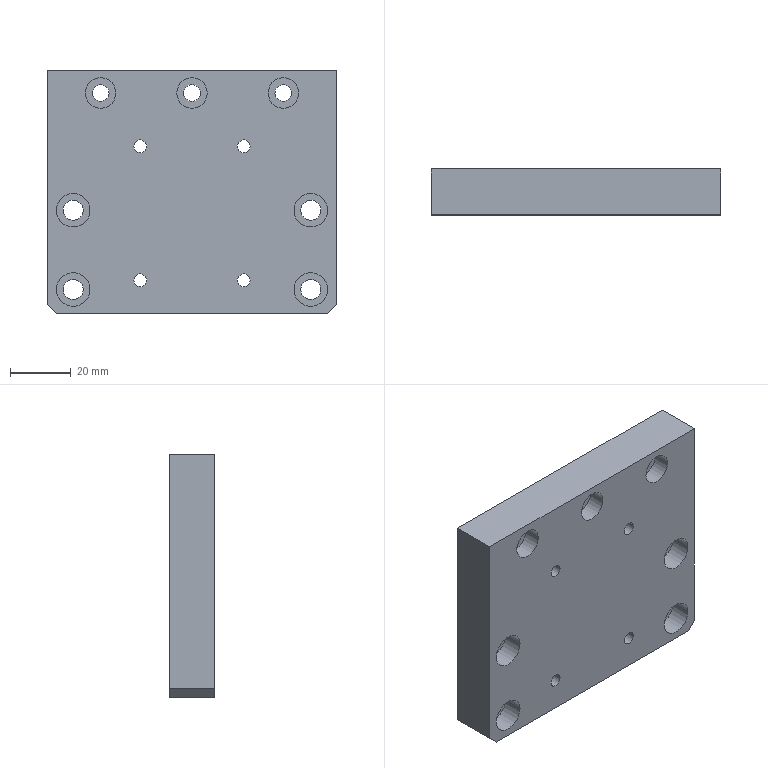Component | SolidWorks | LongSideClampingAssemblyBGeneralAssembly-1_FrameLowerPressPlateB-0510-1 | 1 solid | 51 faces | box 95 x 15 x 80 mm | volume 107321 mm3 | cylinder 36 | plane 15 | commonest cylinder face diameters 4.2 x8 11 x8 6.6 x8 10 x6 5.5 x6 | material Q235-A
build123d program:
from build123d import *

# Parameters (mm, degrees)
SKETCH1_W                                          = 95
SKETCH1_H                                          = 80
BOSS_EXTRUDE1_DEPTH                                = 15
CHAMFER1_SIZE                                      = 3
HOLE_SIZE_ACCORDING_TO_TYPE_OF_HEX_SOC_D           = 6.6
HOLE_SIZE_ACCORDING_TO_TYPE_OF_HEX_SOC_CBORE_D     = 11
HOLE_SIZE_ACCORDING_TO_TYPE_OF_HEX_SOC_CBORE_DEPTH = 6.8
M5_TAPPED_HOLE1_D                                  = 4.2
HOLE_SIZE_ACCORDING_TO_TYPE_OF_HEX_2_D             = 5.5
HOLE_SIZE_ACCORDING_TO_TYPE_OF_HEX_2_CBORE_D       = 10
HOLE_SIZE_ACCORDING_TO_TYPE_OF_HEX_2_CBORE_DEPTH   = 5.7


with BuildPart() as part:
    # Sketch1 → Boss-Extrude1 (new body)
    with BuildSketch(Plane.XY):
        with Locations((-47.5, 40)):
            Rectangle(SKETCH1_W, SKETCH1_H)
    extrude(amount=BOSS_EXTRUDE1_DEPTH)

    # Chamfer1
    chamfer1_edges = [part.edges().sort_by_distance(p)[0] for p in [
        (0, 0, 7.5),
        (-95, 0, 7.5),
    ]]
    chamfer(chamfer1_edges, length=CHAMFER1_SIZE)

    # Hole Size _According to_ Type of Hex Soc (through all)
    with Locations(Plane.XY.offset(15)):
        with Locations((-8.5, 8), (-86.5, 8), (-8.5, 34), (-86.5, 34)):
            CounterBoreHole(HOLE_SIZE_ACCORDING_TO_TYPE_OF_HEX_SOC_D / 2, HOLE_SIZE_ACCORDING_TO_TYPE_OF_HEX_SOC_CBORE_D / 2, HOLE_SIZE_ACCORDING_TO_TYPE_OF_HEX_SOC_CBORE_DEPTH)

    # M5 Tapped Hole1 (through all)
    with Locations(Plane.XY.offset(15)):
        with Locations((-64.5, 55), (-30.5, 55), (-64.5, 11), (-30.5, 11)):
            Hole(M5_TAPPED_HOLE1_D / 2)

    # Hole Size _According to_ Type of Hex 2 (through all)
    with Locations(Plane.XY.offset(15)):
        with Locations((-47.5, 72.5), (-77.5, 72.5), (-17.5, 72.5)):
            CounterBoreHole(HOLE_SIZE_ACCORDING_TO_TYPE_OF_HEX_2_D / 2, HOLE_SIZE_ACCORDING_TO_TYPE_OF_HEX_2_CBORE_D / 2, HOLE_SIZE_ACCORDING_TO_TYPE_OF_HEX_2_CBORE_DEPTH)


solid = part.part

# Placed as in the assembly
solid = solid.moved(Location((-3073.158, -127.609, 3497.5), (90, 0, 0)))